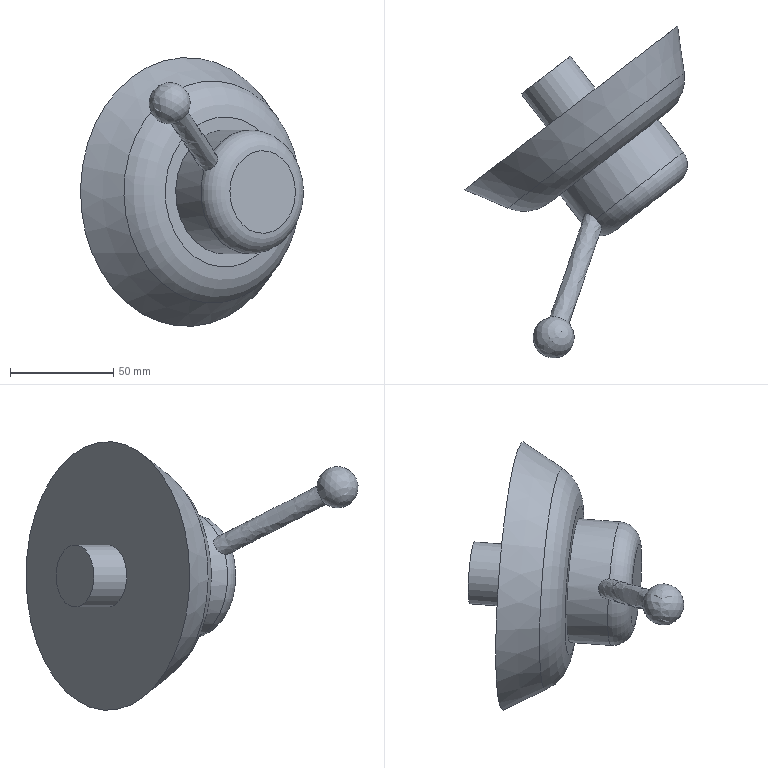Component | NX | BANSHOU2_2 | 1 solid | 11 faces | box 107.87 x 160.69 x 130 mm | volume 400459 mm3 | plane 4 | cylinder 2 | torus 2 | cone 1 | spline 1 | sphere 1 | commonest cylinder face diameters 30 x1 60 x1
STEP:
#1=CARTESIAN_POINT('',(0.,0.,0.));
#2=DIRECTION('',(0.,0.,1.));
#3=DIRECTION('',(1.,0.,0.));
#4=AXIS2_PLACEMENT_3D('',#1,#2,#3);
#5=CARTESIAN_POINT('',(170.195,-134.077,-526.));
#6=VERTEX_POINT('',#5);
#7=CARTESIAN_POINT('',(156.458,-144.627,-516.));
#8=DIRECTION('',(0.6091,-0.7931,0.));
#9=DIRECTION('',(0.6869,0.5275,-0.5));
#10=AXIS2_PLACEMENT_3D('',#7,#8,#9);
#11=CIRCLE('',#10,20.);
#12=CARTESIAN_POINT('',(170.195,-134.077,-526.));
#13=DIRECTION('',(-0.6091,0.7931,-0.));
#14=DIRECTION('',(-0.6869,-0.5275,0.5));
#15=AXIS2_PLACEMENT_3D('',#12,#13,#14);
#16=PLANE('',#15);
#17=CARTESIAN_POINT('',(-0.,-0.));
#18=CARTESIAN_POINT('',(-0.,34.641));
#19=CARTESIAN_POINT('',(30.,17.321));
#20=CARTESIAN_POINT('',(60.,0.));
#21=CARTESIAN_POINT('',(30.,-17.321));
#22=CARTESIAN_POINT('',(-0.,-34.641));
#23=CARTESIAN_POINT('',(-0.,-0.));
#24=(BOUNDED_CURVE()B_SPLINE_CURVE(2,(#17,#18,#19,#20,#21,#22,#23),.UNSPECIFIED.,.T.,.F.)B_SPLINE_CURVE_WITH_KNOTS((1,2,2,2,2,1),(-2.094,0.,2.094,4.189,6.283,8.378),.UNSPECIFIED.)CURVE()GEOMETRIC_REPRESENTATION_ITEM()RATIONAL_B_SPLINE_CURVE((1.,0.5,1.,0.5,1.,0.5,1.))REPRESENTATION_ITEM(''));
#25=(GEOMETRIC_REPRESENTATION_CONTEXT(2)PARAMETRIC_REPRESENTATION_CONTEXT()REPRESENTATION_CONTEXT('',''));
#26=DEFINITIONAL_REPRESENTATION('',(#24),#25);
#27=PCURVE('',#16,#26);
#28=CARTESIAN_POINT('',(150.367,-136.696,-516.));
#29=DIRECTION('',(0.6091,-0.7931,0.));
#30=DIRECTION('',(0.6869,0.5275,-0.5));
#31=AXIS2_PLACEMENT_3D('',#28,#29,#30);
#32=TOROIDAL_SURFACE('',#31,20.,10.);
#33=CARTESIAN_POINT('',(0.,7.854));
#34=DIRECTION('',(1.,0.));
#35=VECTOR('',#34,1.);
#36=LINE('',#33,#35);
#37=(GEOMETRIC_REPRESENTATION_CONTEXT(2)PARAMETRIC_REPRESENTATION_CONTEXT()REPRESENTATION_CONTEXT('',''));
#38=DEFINITIONAL_REPRESENTATION('',(#36),#37);
#39=PCURVE('',#32,#38);
#40=SURFACE_CURVE('',#11,(#27,#39),.PCURVE_S1.);
#41=EDGE_CURVE('',#6,#6,#40,.T.);
#42=ORIENTED_EDGE('',*,*,#41,.T.);
#43=EDGE_LOOP('',(#42));
#44=FACE_BOUND('',#43,.T.);
#45=ADVANCED_FACE('',(#44),#16,.F.);
#46=CARTESIAN_POINT('',(118.035,-73.266,-523.5));
#47=VERTEX_POINT('',#46);
#48=CARTESIAN_POINT('',(107.732,-81.178,-516.));
#49=DIRECTION('',(0.6091,-0.7931,0.));
#50=DIRECTION('',(0.6869,0.5275,-0.5));
#51=AXIS2_PLACEMENT_3D('',#48,#49,#50);
#52=CIRCLE('',#51,15.);
#53=CARTESIAN_POINT('',(107.732,-81.178,-516.));
#54=DIRECTION('',(0.6091,-0.7931,0.));
#55=DIRECTION('',(0.6869,0.5275,-0.5));
#56=AXIS2_PLACEMENT_3D('',#53,#54,#55);
#57=PLANE('',#56);
#58=CARTESIAN_POINT('',(0.,0.));
#59=DIRECTION('',(1.,-0.));
#60=AXIS2_PLACEMENT_2D('',#58,#59);
#61=CIRCLE('',#60,15.);
#62=(GEOMETRIC_REPRESENTATION_CONTEXT(2)PARAMETRIC_REPRESENTATION_CONTEXT()REPRESENTATION_CONTEXT('',''));
#63=DEFINITIONAL_REPRESENTATION('',(#61),#62);
#64=PCURVE('',#57,#63);
#65=CARTESIAN_POINT('',(119.913,-97.04,-516.));
#66=DIRECTION('',(0.6091,-0.7931,0.));
#67=DIRECTION('',(0.6869,0.5275,-0.5));
#68=AXIS2_PLACEMENT_3D('',#65,#66,#67);
#69=CYLINDRICAL_SURFACE('',#68,15.);
#70=CARTESIAN_POINT('',(0.,-20.));
#71=DIRECTION('',(1.,0.));
#72=VECTOR('',#71,1.);
#73=LINE('',#70,#72);
#74=(GEOMETRIC_REPRESENTATION_CONTEXT(2)PARAMETRIC_REPRESENTATION_CONTEXT()REPRESENTATION_CONTEXT('',''));
#75=DEFINITIONAL_REPRESENTATION('',(#73),#74);
#76=PCURVE('',#69,#75);
#77=SURFACE_CURVE('',#52,(#64,#76),.PCURVE_S1.);
#78=EDGE_CURVE('',#47,#47,#77,.T.);
#79=ORIENTED_EDGE('',*,*,#78,.F.);
#80=EDGE_LOOP('',(#79));
#81=FACE_BOUND('',#80,.T.);
#82=ADVANCED_FACE('',(#81),#57,.F.);
#83=CARTESIAN_POINT('',(130.216,-89.128,-523.5));
#84=VERTEX_POINT('',#83);
#85=CARTESIAN_POINT('',(119.913,-97.04,-516.));
#86=DIRECTION('',(0.6091,-0.7931,0.));
#87=DIRECTION('',(0.6869,0.5275,-0.5));
#88=AXIS2_PLACEMENT_3D('',#85,#86,#87);
#89=CIRCLE('',#88,15.);
#90=CARTESIAN_POINT('',(0.,0.));
#91=DIRECTION('',(1.,0.));
#92=VECTOR('',#91,1.);
#93=LINE('',#90,#92);
#94=(GEOMETRIC_REPRESENTATION_CONTEXT(2)PARAMETRIC_REPRESENTATION_CONTEXT()REPRESENTATION_CONTEXT('',''));
#95=DEFINITIONAL_REPRESENTATION('',(#93),#94);
#96=PCURVE('',#69,#95);
#97=CARTESIAN_POINT('',(130.216,-89.128,-523.5));
#98=DIRECTION('',(0.6091,-0.7931,0.));
#99=DIRECTION('',(0.6869,0.5275,-0.5));
#100=AXIS2_PLACEMENT_3D('',#97,#98,#99);
#101=PLANE('',#100);
#102=CARTESIAN_POINT('',(-15.,0.));
#103=DIRECTION('',(1.,-0.));
#104=AXIS2_PLACEMENT_2D('',#102,#103);
#105=CIRCLE('',#104,15.);
#106=(GEOMETRIC_REPRESENTATION_CONTEXT(2)PARAMETRIC_REPRESENTATION_CONTEXT()REPRESENTATION_CONTEXT('',''));
#107=DEFINITIONAL_REPRESENTATION('',(#105),#106);
#108=PCURVE('',#101,#107);
#109=SURFACE_CURVE('',#89,(#96,#108),.PCURVE_S1.);
#110=EDGE_CURVE('',#84,#84,#109,.T.);
#111=ORIENTED_EDGE('',*,*,#110,.F.);
#112=CARTESIAN_POINT('',(118.035,-73.266,-523.5));
#113=CARTESIAN_POINT('',(130.216,-89.128,-523.5));
#114=B_SPLINE_CURVE_WITH_KNOTS('',1,(#112,#113),.UNSPECIFIED.,.F.,.F.,(2,2),(-20.,0.),.PIECEWISE_BEZIER_KNOTS.);
#115=CARTESIAN_POINT('',(0.,0.));
#116=DIRECTION('',(0.,1.));
#117=VECTOR('',#116,1.);
#118=LINE('',#115,#117);
#119=(GEOMETRIC_REPRESENTATION_CONTEXT(2)PARAMETRIC_REPRESENTATION_CONTEXT()REPRESENTATION_CONTEXT('',''));
#120=DEFINITIONAL_REPRESENTATION('',(#118),#119);
#121=PCURVE('',#69,#120);
#122=CARTESIAN_POINT('',(6.283,0.));
#123=DIRECTION('',(0.,1.));
#124=VECTOR('',#123,1.);
#125=LINE('',#122,#124);
#126=(GEOMETRIC_REPRESENTATION_CONTEXT(2)PARAMETRIC_REPRESENTATION_CONTEXT()REPRESENTATION_CONTEXT('',''));
#127=DEFINITIONAL_REPRESENTATION('',(#125),#126);
#128=PCURVE('',#69,#127);
#129=SEAM_CURVE('',#114,(#121,#128),.PCURVE_S1.);
#130=EDGE_CURVE('',#47,#84,#129,.T.);
#131=ORIENTED_EDGE('',*,*,#130,.F.);
#132=ORIENTED_EDGE('',*,*,#78,.T.);
#133=ORIENTED_EDGE('',*,*,#130,.T.);
#134=EDGE_LOOP('',(#111,#131,#132,#133));
#135=FACE_BOUND('',#134,.T.);
#136=ADVANCED_FACE('',(#135),#69,.T.);
#137=CARTESIAN_POINT('',(164.559,-62.754,-548.5));
#138=VERTEX_POINT('',#137);
#139=CARTESIAN_POINT('',(119.913,-97.04,-516.));
#140=DIRECTION('',(0.6091,-0.7931,0.));
#141=DIRECTION('',(0.6869,0.5275,-0.5));
#142=AXIS2_PLACEMENT_3D('',#139,#140,#141);
#143=CIRCLE('',#142,65.);
#144=CARTESIAN_POINT('',(-15.,0.));
#145=DIRECTION('',(1.,0.));
#146=AXIS2_PLACEMENT_2D('',#144,#145);
#147=CIRCLE('',#146,65.);
#148=(GEOMETRIC_REPRESENTATION_CONTEXT(2)PARAMETRIC_REPRESENTATION_CONTEXT()REPRESENTATION_CONTEXT('',''));
#149=DEFINITIONAL_REPRESENTATION('',(#147),#148);
#150=PCURVE('',#101,#149);
#151=CARTESIAN_POINT('',(119.913,-97.04,-516.));
#152=DIRECTION('',(-0.6091,0.7931,-0.));
#153=DIRECTION('',(-0.6869,-0.5275,0.5));
#154=AXIS2_PLACEMENT_3D('',#151,#152,#153);
#155=CONICAL_SURFACE('',#154,65.,0.5155);
#156=CARTESIAN_POINT('',(9.425,0.));
#157=DIRECTION('',(-1.,0.));
#158=VECTOR('',#157,1.);
#159=LINE('',#156,#158);
#160=(GEOMETRIC_REPRESENTATION_CONTEXT(2)PARAMETRIC_REPRESENTATION_CONTEXT()REPRESENTATION_CONTEXT('',''));
#161=DEFINITIONAL_REPRESENTATION('',(#159),#160);
#162=PCURVE('',#155,#161);
#163=SURFACE_CURVE('',#143,(#150,#162),.PCURVE_S1.);
#164=EDGE_CURVE('',#138,#138,#163,.T.);
#165=ORIENTED_EDGE('',*,*,#164,.F.);
#166=EDGE_LOOP('',(#165));
#167=FACE_BOUND('',#166,.T.);
#168=ORIENTED_EDGE('',*,*,#110,.T.);
#169=EDGE_LOOP('',(#168));
#170=FACE_BOUND('',#169,.T.);
#171=ADVANCED_FACE('',(#167,#170),#101,.F.);
#172=CARTESIAN_POINT('',(168.925,-84.442,-542.873));
#173=VERTEX_POINT('',#172);
#174=CARTESIAN_POINT('',(132.01,-112.792,-516.));
#175=DIRECTION('',(0.6091,-0.7931,0.));
#176=DIRECTION('',(0.6869,0.5275,-0.5));
#177=AXIS2_PLACEMENT_3D('',#174,#175,#176);
#178=CIRCLE('',#177,53.746);
#179=CARTESIAN_POINT('',(9.425,-19.86));
#180=DIRECTION('',(-1.,0.));
#181=VECTOR('',#180,1.);
#182=LINE('',#179,#181);
#183=(GEOMETRIC_REPRESENTATION_CONTEXT(2)PARAMETRIC_REPRESENTATION_CONTEXT()REPRESENTATION_CONTEXT('',''));
#184=DEFINITIONAL_REPRESENTATION('',(#182),#183);
#185=PCURVE('',#155,#184);
#186=CARTESIAN_POINT('',(126.004,-104.971,-516.));
#187=DIRECTION('',(0.6091,-0.7931,0.));
#188=DIRECTION('',(0.6869,0.5275,-0.5));
#189=AXIS2_PLACEMENT_3D('',#186,#187,#188);
#190=TOROIDAL_SURFACE('',#189,36.345,20.);
#191=CARTESIAN_POINT('',(0.,6.799));
#192=DIRECTION('',(1.,0.));
#193=VECTOR('',#192,1.);
#194=LINE('',#191,#193);
#195=(GEOMETRIC_REPRESENTATION_CONTEXT(2)PARAMETRIC_REPRESENTATION_CONTEXT()REPRESENTATION_CONTEXT('',''));
#196=DEFINITIONAL_REPRESENTATION('',(#194),#195);
#197=PCURVE('',#190,#196);
#198=SURFACE_CURVE('',#178,(#185,#197),.PCURVE_S1.);
#199=EDGE_CURVE('',#173,#173,#198,.T.);
#200=ORIENTED_EDGE('',*,*,#199,.F.);
#201=CARTESIAN_POINT('',(168.925,-84.442,-542.873));
#202=CARTESIAN_POINT('',(164.559,-62.754,-548.5));
#203=B_SPLINE_CURVE_WITH_KNOTS('',1,(#201,#202),.UNSPECIFIED.,.F.,.F.,(2,2),(-22.827,0.),.PIECEWISE_BEZIER_KNOTS.);
#204=CARTESIAN_POINT('',(9.425,0.));
#205=DIRECTION('',(0.,1.));
#206=VECTOR('',#205,1.);
#207=LINE('',#204,#206);
#208=(GEOMETRIC_REPRESENTATION_CONTEXT(2)PARAMETRIC_REPRESENTATION_CONTEXT()REPRESENTATION_CONTEXT('',''));
#209=DEFINITIONAL_REPRESENTATION('',(#207),#208);
#210=PCURVE('',#155,#209);
#211=CARTESIAN_POINT('',(3.142,0.));
#212=DIRECTION('',(0.,1.));
#213=VECTOR('',#212,1.);
#214=LINE('',#211,#213);
#215=(GEOMETRIC_REPRESENTATION_CONTEXT(2)PARAMETRIC_REPRESENTATION_CONTEXT()REPRESENTATION_CONTEXT('',''));
#216=DEFINITIONAL_REPRESENTATION('',(#214),#215);
#217=PCURVE('',#155,#216);
#218=SEAM_CURVE('',#203,(#210,#217),.PCURVE_S1.);
#219=EDGE_CURVE('',#173,#138,#218,.T.);
#220=ORIENTED_EDGE('',*,*,#219,.T.);
#221=ORIENTED_EDGE('',*,*,#164,.T.);
#222=ORIENTED_EDGE('',*,*,#219,.F.);
#223=EDGE_LOOP('',(#200,#220,#221,#222));
#224=FACE_BOUND('',#223,.T.);
#225=ADVANCED_FACE('',(#224),#155,.T.);
#226=CARTESIAN_POINT('',(163.15,-101.662,-534.173));
#227=VERTEX_POINT('',#226);
#228=CARTESIAN_POINT('',(138.186,-120.834,-516.));
#229=DIRECTION('',(0.6091,-0.7931,0.));
#230=DIRECTION('',(0.6869,0.5275,-0.5));
#231=AXIS2_PLACEMENT_3D('',#228,#229,#230);
#232=CIRCLE('',#231,36.345);
#233=CARTESIAN_POINT('',(0.,7.854));
#234=DIRECTION('',(1.,0.));
#235=VECTOR('',#234,1.);
#236=LINE('',#233,#235);
#237=(GEOMETRIC_REPRESENTATION_CONTEXT(2)PARAMETRIC_REPRESENTATION_CONTEXT()REPRESENTATION_CONTEXT('',''));
#238=DEFINITIONAL_REPRESENTATION('',(#236),#237);
#239=PCURVE('',#190,#238);
#240=CARTESIAN_POINT('',(163.15,-101.662,-534.173));
#241=DIRECTION('',(-0.6091,0.7931,-0.));
#242=DIRECTION('',(-0.6869,-0.5275,0.5));
#243=AXIS2_PLACEMENT_3D('',#240,#241,#242);
#244=PLANE('',#243);
#245=CARTESIAN_POINT('',(-0.,0.));
#246=CARTESIAN_POINT('',(-0.,62.952));
#247=CARTESIAN_POINT('',(54.518,31.476));
#248=CARTESIAN_POINT('',(109.036,0.));
#249=CARTESIAN_POINT('',(54.518,-31.476));
#250=CARTESIAN_POINT('',(-0.,-62.952));
#251=CARTESIAN_POINT('',(-0.,0.));
#252=(BOUNDED_CURVE()B_SPLINE_CURVE(2,(#245,#246,#247,#248,#249,#250,#251),.UNSPECIFIED.,.T.,.F.)B_SPLINE_CURVE_WITH_KNOTS((1,2,2,2,2,1),(-2.094,0.,2.094,4.189,6.283,8.378),.UNSPECIFIED.)CURVE()GEOMETRIC_REPRESENTATION_ITEM()RATIONAL_B_SPLINE_CURVE((1.,0.5,1.,0.5,1.,0.5,1.))REPRESENTATION_ITEM(''));
#253=(GEOMETRIC_REPRESENTATION_CONTEXT(2)PARAMETRIC_REPRESENTATION_CONTEXT()REPRESENTATION_CONTEXT('',''));
#254=DEFINITIONAL_REPRESENTATION('',(#252),#253);
#255=PCURVE('',#244,#254);
#256=SURFACE_CURVE('',#232,(#239,#255),.PCURVE_S1.);
#257=EDGE_CURVE('',#227,#227,#256,.T.);
#258=ORIENTED_EDGE('',*,*,#257,.F.);
#259=CARTESIAN_POINT('',(168.925,-84.442,-542.873));
#260=CARTESIAN_POINT('',(169.605,-87.815,-541.998));
#261=CARTESIAN_POINT('',(169.599,-91.201,-540.805));
#262=CARTESIAN_POINT('',(168.901,-94.43,-539.349));
#263=CARTESIAN_POINT('',(167.54,-97.34,-537.703));
#264=CARTESIAN_POINT('',(165.588,-99.789,-535.948));
#265=CARTESIAN_POINT('',(163.15,-101.662,-534.173));
#266=(BOUNDED_CURVE()B_SPLINE_CURVE(6,(#259,#260,#261,#262,#263,#264,#265),.UNSPECIFIED.,.F.,.F.)B_SPLINE_CURVE_WITH_KNOTS((7,7),(0.5155,1.571),.PIECEWISE_BEZIER_KNOTS.)CURVE()GEOMETRIC_REPRESENTATION_ITEM()RATIONAL_B_SPLINE_CURVE((1.014,1.005,0.9991,0.9972,0.9991,1.005,1.014))REPRESENTATION_ITEM(''));
#267=CARTESIAN_POINT('',(0.,6.283));
#268=DIRECTION('',(0.,1.));
#269=VECTOR('',#268,1.);
#270=LINE('',#267,#269);
#271=(GEOMETRIC_REPRESENTATION_CONTEXT(2)PARAMETRIC_REPRESENTATION_CONTEXT()REPRESENTATION_CONTEXT('',''));
#272=DEFINITIONAL_REPRESENTATION('',(#270),#271);
#273=PCURVE('',#190,#272);
#274=CARTESIAN_POINT('',(6.283,6.283));
#275=DIRECTION('',(0.,1.));
#276=VECTOR('',#275,1.);
#277=LINE('',#274,#276);
#278=(GEOMETRIC_REPRESENTATION_CONTEXT(2)PARAMETRIC_REPRESENTATION_CONTEXT()REPRESENTATION_CONTEXT('',''));
#279=DEFINITIONAL_REPRESENTATION('',(#277),#278);
#280=PCURVE('',#190,#279);
#281=SEAM_CURVE('',#266,(#273,#280),.PCURVE_S1.);
#282=EDGE_CURVE('',#173,#227,#281,.T.);
#283=ORIENTED_EDGE('',*,*,#282,.F.);
#284=ORIENTED_EDGE('',*,*,#199,.T.);
#285=ORIENTED_EDGE('',*,*,#282,.T.);
#286=EDGE_LOOP('',(#258,#283,#284,#285));
#287=FACE_BOUND('',#286,.T.);
#288=ADVANCED_FACE('',(#287),#190,.T.);
#289=CARTESIAN_POINT('',(158.791,-105.009,-531.));
#290=VERTEX_POINT('',#289);
#291=CARTESIAN_POINT('',(138.186,-120.834,-516.));
#292=DIRECTION('',(0.6091,-0.7931,0.));
#293=DIRECTION('',(0.6869,0.5275,-0.5));
#294=AXIS2_PLACEMENT_3D('',#291,#292,#293);
#295=CIRCLE('',#294,30.);
#296=CARTESIAN_POINT('',(6.345,0.));
#297=CARTESIAN_POINT('',(6.345,51.962));
#298=CARTESIAN_POINT('',(51.345,25.981));
#299=CARTESIAN_POINT('',(96.345,0.));
#300=CARTESIAN_POINT('',(51.345,-25.981));
#301=CARTESIAN_POINT('',(6.345,-51.962));
#302=CARTESIAN_POINT('',(6.345,0.));
#303=(BOUNDED_CURVE()B_SPLINE_CURVE(2,(#296,#297,#298,#299,#300,#301,#302),.UNSPECIFIED.,.T.,.F.)B_SPLINE_CURVE_WITH_KNOTS((1,2,2,2,2,1),(-2.094,0.,2.094,4.189,6.283,8.378),.UNSPECIFIED.)CURVE()GEOMETRIC_REPRESENTATION_ITEM()RATIONAL_B_SPLINE_CURVE((1.,0.5,1.,0.5,1.,0.5,1.))REPRESENTATION_ITEM(''));
#304=(GEOMETRIC_REPRESENTATION_CONTEXT(2)PARAMETRIC_REPRESENTATION_CONTEXT()REPRESENTATION_CONTEXT('',''));
#305=DEFINITIONAL_REPRESENTATION('',(#303),#304);
#306=PCURVE('',#244,#305);
#307=CARTESIAN_POINT('',(119.913,-97.04,-516.));
#308=DIRECTION('',(0.6091,-0.7931,0.));
#309=DIRECTION('',(0.6869,0.5275,-0.5));
#310=AXIS2_PLACEMENT_3D('',#307,#308,#309);
#311=CYLINDRICAL_SURFACE('',#310,30.);
#312=CARTESIAN_POINT('',(0.,30.));
#313=DIRECTION('',(1.,0.));
#314=VECTOR('',#313,1.);
#315=LINE('',#312,#314);
#316=(GEOMETRIC_REPRESENTATION_CONTEXT(2)PARAMETRIC_REPRESENTATION_CONTEXT()REPRESENTATION_CONTEXT('',''));
#317=DEFINITIONAL_REPRESENTATION('',(#315),#316);
#318=PCURVE('',#311,#317);
#319=SURFACE_CURVE('',#295,(#306,#318),.PCURVE_S1.);
#320=EDGE_CURVE('',#290,#290,#319,.T.);
#321=ORIENTED_EDGE('',*,*,#320,.F.);
#322=EDGE_LOOP('',(#321));
#323=FACE_BOUND('',#322,.T.);
#324=ORIENTED_EDGE('',*,*,#257,.T.);
#325=EDGE_LOOP('',(#324));
#326=FACE_BOUND('',#325,.T.);
#327=ADVANCED_FACE('',(#323,#326),#244,.F.);
#328=CARTESIAN_POINT('',(170.973,-120.872,-531.));
#329=VERTEX_POINT('',#328);
#330=CARTESIAN_POINT('',(132.021,-150.784,-496.896));
#331=VERTEX_POINT('',#330);
#332=CARTESIAN_POINT('',(150.367,-136.696,-516.));
#333=DIRECTION('',(0.6091,-0.7931,0.));
#334=DIRECTION('',(0.6869,0.5275,-0.5));
#335=AXIS2_PLACEMENT_3D('',#332,#333,#334);
#336=CIRCLE('',#335,30.);
#337=CARTESIAN_POINT('',(-6.283,50.));
#338=DIRECTION('',(1.,0.));
#339=VECTOR('',#338,1.);
#340=LINE('',#337,#339);
#341=(GEOMETRIC_REPRESENTATION_CONTEXT(2)PARAMETRIC_REPRESENTATION_CONTEXT()REPRESENTATION_CONTEXT('',''));
#342=DEFINITIONAL_REPRESENTATION('',(#340),#341);
#343=PCURVE('',#311,#342);
#344=CARTESIAN_POINT('',(-6.283,6.283));
#345=DIRECTION('',(1.,0.));
#346=VECTOR('',#345,1.);
#347=LINE('',#344,#346);
#348=(GEOMETRIC_REPRESENTATION_CONTEXT(2)PARAMETRIC_REPRESENTATION_CONTEXT()REPRESENTATION_CONTEXT('',''));
#349=DEFINITIONAL_REPRESENTATION('',(#347),#348);
#350=PCURVE('',#32,#349);
#351=SURFACE_CURVE('',#336,(#343,#350),.PCURVE_S1.);
#352=EDGE_CURVE('',#329,#331,#351,.T.);
#353=ORIENTED_EDGE('',*,*,#352,.F.);
#354=CARTESIAN_POINT('',(158.791,-105.009,-531.));
#355=CARTESIAN_POINT('',(170.973,-120.872,-531.));
#356=B_SPLINE_CURVE_WITH_KNOTS('',1,(#354,#355),.UNSPECIFIED.,.F.,.F.,(2,2),(30.,50.),.PIECEWISE_BEZIER_KNOTS.);
#357=CARTESIAN_POINT('',(0.,0.));
#358=DIRECTION('',(0.,1.));
#359=VECTOR('',#358,1.);
#360=LINE('',#357,#359);
#361=(GEOMETRIC_REPRESENTATION_CONTEXT(2)PARAMETRIC_REPRESENTATION_CONTEXT()REPRESENTATION_CONTEXT('',''));
#362=DEFINITIONAL_REPRESENTATION('',(#360),#361);
#363=PCURVE('',#311,#362);
#364=CARTESIAN_POINT('',(6.283,0.));
#365=DIRECTION('',(0.,1.));
#366=VECTOR('',#365,1.);
#367=LINE('',#364,#366);
#368=(GEOMETRIC_REPRESENTATION_CONTEXT(2)PARAMETRIC_REPRESENTATION_CONTEXT()REPRESENTATION_CONTEXT('',''));
#369=DEFINITIONAL_REPRESENTATION('',(#367),#368);
#370=PCURVE('',#311,#369);
#371=SEAM_CURVE('',#356,(#363,#370),.PCURVE_S1.);
#372=EDGE_CURVE('',#290,#329,#371,.T.);
#373=ORIENTED_EDGE('',*,*,#372,.F.);
#374=ORIENTED_EDGE('',*,*,#320,.T.);
#375=ORIENTED_EDGE('',*,*,#372,.T.);
#376=CARTESIAN_POINT('',(128.073,-153.817,-505.52));
#377=VERTEX_POINT('',#376);
#378=CARTESIAN_POINT('',(150.367,-136.696,-516.));
#379=DIRECTION('',(0.6091,-0.7931,0.));
#380=DIRECTION('',(0.6869,0.5275,-0.5));
#381=AXIS2_PLACEMENT_3D('',#378,#379,#380);
#382=CIRCLE('',#381,30.);
#383=CARTESIAN_POINT('',(0.,50.));
#384=DIRECTION('',(1.,0.));
#385=VECTOR('',#384,1.);
#386=LINE('',#383,#385);
#387=(GEOMETRIC_REPRESENTATION_CONTEXT(2)PARAMETRIC_REPRESENTATION_CONTEXT()REPRESENTATION_CONTEXT('',''));
#388=DEFINITIONAL_REPRESENTATION('',(#386),#387);
#389=PCURVE('',#311,#388);
#390=CARTESIAN_POINT('',(-0.,6.283));
#391=DIRECTION('',(1.,0.));
#392=VECTOR('',#391,1.);
#393=LINE('',#390,#392);
#394=(GEOMETRIC_REPRESENTATION_CONTEXT(2)PARAMETRIC_REPRESENTATION_CONTEXT()REPRESENTATION_CONTEXT('',''));
#395=DEFINITIONAL_REPRESENTATION('',(#393),#394);
#396=PCURVE('',#32,#395);
#397=SURFACE_CURVE('',#382,(#389,#396),.PCURVE_S1.);
#398=EDGE_CURVE('',#377,#329,#397,.T.);
#399=ORIENTED_EDGE('',*,*,#398,.F.);
#400=CARTESIAN_POINT('',(128.073,-153.817,-505.52));
#401=CARTESIAN_POINT('',(127.309,-152.761,-505.419));
#402=CARTESIAN_POINT('',(126.684,-151.667,-504.941));
#403=CARTESIAN_POINT('',(126.105,-149.738,-503.283));
#404=CARTESIAN_POINT('',(126.199,-148.955,-502.134));
#405=CARTESIAN_POINT('',(127.226,-148.16,-499.883));
#406=CARTESIAN_POINT('',(128.145,-148.167,-498.822));
#407=CARTESIAN_POINT('',(130.132,-148.991,-497.378));
#408=CARTESIAN_POINT('',(131.173,-149.792,-496.979));
#409=CARTESIAN_POINT('',(132.021,-150.784,-496.896));
#410=B_SPLINE_CURVE_WITH_KNOTS('',3,(#400,#401,#402,#403,#404,#405,#406,#407,#408,#409),.UNSPECIFIED.,.F.,.F.,(4,2,2,2,4),(0.,0.25,0.5,0.75,1.),.UNSPECIFIED.);
#411=CARTESIAN_POINT('',(3.308,50.));
#412=CARTESIAN_POINT('',(3.308,49.763));
#413=CARTESIAN_POINT('',(3.305,49.293));
#414=CARTESIAN_POINT('',(3.3,48.608));
#415=CARTESIAN_POINT('',(3.291,47.952));
#416=CARTESIAN_POINT('',(3.28,47.333));
#417=CARTESIAN_POINT('',(3.266,46.763));
#418=CARTESIAN_POINT('',(3.25,46.247));
#419=CARTESIAN_POINT('',(3.231,45.811));
#420=CARTESIAN_POINT('',(3.21,45.46));
#421=CARTESIAN_POINT('',(3.188,45.2));
#422=CARTESIAN_POINT('',(3.165,45.039));
#423=CARTESIAN_POINT('',(3.142,44.981));
#424=CARTESIAN_POINT('',(3.118,45.036));
#425=CARTESIAN_POINT('',(3.095,45.197));
#426=CARTESIAN_POINT('',(3.073,45.455));
#427=CARTESIAN_POINT('',(3.053,45.805));
#428=CARTESIAN_POINT('',(3.034,46.237));
#429=CARTESIAN_POINT('',(3.018,46.747));
#430=CARTESIAN_POINT('',(3.004,47.318));
#431=CARTESIAN_POINT('',(2.992,47.94));
#432=CARTESIAN_POINT('',(2.984,48.601));
#433=CARTESIAN_POINT('',(2.978,49.291));
#434=CARTESIAN_POINT('',(2.976,49.763));
#435=CARTESIAN_POINT('',(2.975,50.));
#436=B_SPLINE_CURVE_WITH_KNOTS('',3,(#411,#412,#413,#414,#415,#416,#417,#418,#419,#420,#421,#422,#423,#424,#425,#426,#427,#428,#429,#430,#431,#432,#433,#434,#435),.UNSPECIFIED.,.F.,.F.,(4,1,1,1,1,1,1,1,1,1,1,1,1,1,1,1,1,1,1,1,1,1,4),(0.,0.04545,0.09091,0.1364,0.1818,0.2273,0.2727,0.3182,0.3636,0.4091,0.4545,0.5,0.5455,0.5909,0.6364,0.6818,0.7273,0.7727,0.8182,0.8636,0.9091,0.9545,1.),.QUASI_UNIFORM_KNOTS.);
#437=(GEOMETRIC_REPRESENTATION_CONTEXT(2)PARAMETRIC_REPRESENTATION_CONTEXT()REPRESENTATION_CONTEXT('',''));
#438=DEFINITIONAL_REPRESENTATION('',(#436),#437);
#439=PCURVE('',#311,#438);
#440=CARTESIAN_POINT('',(134.905,-152.793,-505.3));
#441=CARTESIAN_POINT('',(125.04,-181.791,-490.586));
#442=CARTESIAN_POINT('',(115.176,-210.789,-475.872));
#443=CARTESIAN_POINT('',(136.307,-151.717,-502.238));
#444=CARTESIAN_POINT('',(126.442,-180.715,-487.524));
#445=CARTESIAN_POINT('',(116.578,-209.712,-472.81));
#446=CARTESIAN_POINT('',(136.468,-150.628,-499.984));
#447=CARTESIAN_POINT('',(126.604,-179.625,-485.27));
#448=CARTESIAN_POINT('',(116.739,-208.623,-470.555));
#449=CARTESIAN_POINT('',(134.773,-149.365,-498.631));
#450=CARTESIAN_POINT('',(124.909,-178.363,-483.917));
#451=CARTESIAN_POINT('',(115.044,-207.361,-469.203));
#452=CARTESIAN_POINT('',(131.694,-147.869,-497.747));
#453=CARTESIAN_POINT('',(121.83,-176.867,-483.033));
#454=CARTESIAN_POINT('',(111.965,-205.865,-468.319));
#455=CARTESIAN_POINT('',(129.299,-147.144,-497.926));
#456=CARTESIAN_POINT('',(119.434,-176.142,-483.211));
#457=CARTESIAN_POINT('',(109.57,-205.14,-468.497));
#458=CARTESIAN_POINT('',(127.598,-147.485,-499.738));
#459=CARTESIAN_POINT('',(117.733,-176.483,-485.024));
#460=CARTESIAN_POINT('',(107.869,-205.481,-470.31));
#461=CARTESIAN_POINT('',(126.196,-148.562,-502.8));
#462=CARTESIAN_POINT('',(116.331,-177.56,-488.086));
#463=CARTESIAN_POINT('',(106.467,-206.558,-473.372));
#464=CARTESIAN_POINT('',(126.034,-149.651,-505.055));
#465=CARTESIAN_POINT('',(116.17,-178.649,-490.341));
#466=CARTESIAN_POINT('',(106.305,-207.647,-475.627));
#467=CARTESIAN_POINT('',(127.729,-150.914,-506.407));
#468=CARTESIAN_POINT('',(117.864,-179.912,-491.693));
#469=CARTESIAN_POINT('',(108.,-208.91,-476.979));
#470=CARTESIAN_POINT('',(130.808,-152.41,-507.291));
#471=CARTESIAN_POINT('',(120.943,-181.408,-492.577));
#472=CARTESIAN_POINT('',(111.079,-210.406,-477.863));
#473=CARTESIAN_POINT('',(133.204,-153.135,-507.113));
#474=CARTESIAN_POINT('',(123.339,-182.132,-492.399));
#475=CARTESIAN_POINT('',(113.475,-211.13,-477.685));
#476=CARTESIAN_POINT('',(134.905,-152.793,-505.3));
#477=CARTESIAN_POINT('',(125.04,-181.791,-490.586));
#478=CARTESIAN_POINT('',(115.176,-210.789,-475.872));
#479=CARTESIAN_POINT('',(136.307,-151.717,-502.238));
#480=CARTESIAN_POINT('',(126.442,-180.715,-487.524));
#481=CARTESIAN_POINT('',(116.578,-209.712,-472.81));
#482=(BOUNDED_SURFACE()B_SPLINE_SURFACE(4,2,((#440,#441,#442),(#443,#444,#445),(#446,#447,#448),(#449,#450,#451),(#452,#453,#454),(#455,#456,#457),(#458,#459,#460),(#461,#462,#463),(#464,#465,#466),(#467,#468,#469),(#470,#471,#472),(#473,#474,#475),(#476,#477,#478),(#479,#480,#481)),.UNSPECIFIED.,.T.,.F.,.F.)B_SPLINE_SURFACE_WITH_KNOTS((2,3,3,3,3,3,2),(3,3),(-0.25,0.,0.25,0.5,0.75,1.,1.25),(0.,1.),.UNSPECIFIED.)GEOMETRIC_REPRESENTATION_ITEM()RATIONAL_B_SPLINE_SURFACE(((0.5858,0.5858,0.5858),(0.5858,0.5858,0.5858),(0.5523,0.5523,0.5523),(0.5858,0.5858,0.5858),(0.5858,0.5858,0.5858),(0.5523,0.5523,0.5523),(0.5858,0.5858,0.5858),(0.5858,0.5858,0.5858),(0.5523,0.5523,0.5523),(0.5858,0.5858,0.5858),(0.5858,0.5858,0.5858),(0.5523,0.5523,0.5523),(0.5858,0.5858,0.5858),(0.5858,0.5858,0.5858)))REPRESENTATION_ITEM('')SURFACE());
#483=CARTESIAN_POINT('',(0.7339,0.04063));
#484=CARTESIAN_POINT('',(0.7269,0.03893));
#485=CARTESIAN_POINT('',(0.713,0.03562));
#486=CARTESIAN_POINT('',(0.6927,0.03095));
#487=CARTESIAN_POINT('',(0.6727,0.02663));
#488=CARTESIAN_POINT('',(0.6528,0.02269));
#489=CARTESIAN_POINT('',(0.6328,0.01917));
#490=CARTESIAN_POINT('',(0.6123,0.01612));
#491=CARTESIAN_POINT('',(0.5914,0.0136));
#492=CARTESIAN_POINT('',(0.57,0.01163));
#493=CARTESIAN_POINT('',(0.5478,0.01021));
#494=CARTESIAN_POINT('',(0.5249,0.009348));
#495=CARTESIAN_POINT('',(0.5004,0.009053));
#496=CARTESIAN_POINT('',(0.4757,0.009335));
#497=CARTESIAN_POINT('',(0.4527,0.01019));
#498=CARTESIAN_POINT('',(0.4305,0.0116));
#499=CARTESIAN_POINT('',(0.409,0.01356));
#500=CARTESIAN_POINT('',(0.3882,0.01606));
#501=CARTESIAN_POINT('',(0.3678,0.01908));
#502=CARTESIAN_POINT('',(0.3477,0.0226));
#503=CARTESIAN_POINT('',(0.3277,0.02656));
#504=CARTESIAN_POINT('',(0.3076,0.03091));
#505=CARTESIAN_POINT('',(0.2871,0.03561));
#506=CARTESIAN_POINT('',(0.2731,0.03893));
#507=CARTESIAN_POINT('',(0.2661,0.04063));
#508=B_SPLINE_CURVE_WITH_KNOTS('',3,(#483,#484,#485,#486,#487,#488,#489,#490,#491,#492,#493,#494,#495,#496,#497,#498,#499,#500,#501,#502,#503,#504,#505,#506,#507),.UNSPECIFIED.,.F.,.F.,(4,1,1,1,1,1,1,1,1,1,1,1,1,1,1,1,1,1,1,1,1,1,4),(0.,0.04545,0.09091,0.1364,0.1818,0.2273,0.2727,0.3182,0.3636,0.4091,0.4545,0.5,0.5455,0.5909,0.6364,0.6818,0.7273,0.7727,0.8182,0.8636,0.9091,0.9545,1.),.QUASI_UNIFORM_KNOTS.);
#509=(GEOMETRIC_REPRESENTATION_CONTEXT(2)PARAMETRIC_REPRESENTATION_CONTEXT()REPRESENTATION_CONTEXT('',''));
#510=DEFINITIONAL_REPRESENTATION('',(#508),#509);
#511=PCURVE('',#482,#510);
#512=SURFACE_CURVE('',#410,(#439,#511),.PCURVE_S1.);
#513=EDGE_CURVE('',#377,#331,#512,.T.);
#514=ORIENTED_EDGE('',*,*,#513,.T.);
#515=EDGE_LOOP('',(#353,#373,#374,#375,#399,#514));
#516=FACE_BOUND('',#515,.T.);
#517=ADVANCED_FACE('',(#516),#311,.T.);
#518=ORIENTED_EDGE('',*,*,#41,.F.);
#519=CARTESIAN_POINT('',(170.973,-120.872,-531.));
#520=CARTESIAN_POINT('',(172.601,-122.992,-531.));
#521=CARTESIAN_POINT('',(173.603,-125.505,-530.575));
#522=CARTESIAN_POINT('',(173.849,-128.144,-529.76));
#523=CARTESIAN_POINT('',(173.302,-130.62,-528.639));
#524=CARTESIAN_POINT('',(172.031,-132.667,-527.337));
#525=CARTESIAN_POINT('',(170.195,-134.077,-526.));
#526=(BOUNDED_CURVE()B_SPLINE_CURVE(6,(#519,#520,#521,#522,#523,#524,#525),.UNSPECIFIED.,.F.,.F.)B_SPLINE_CURVE_WITH_KNOTS((7,7),(0.,1.571),.PIECEWISE_BEZIER_KNOTS.)CURVE()GEOMETRIC_REPRESENTATION_ITEM()RATIONAL_B_SPLINE_CURVE((1.031,1.01,0.9979,0.994,0.9979,1.01,1.031))REPRESENTATION_ITEM(''));
#527=CARTESIAN_POINT('',(0.,6.283));
#528=DIRECTION('',(0.,1.));
#529=VECTOR('',#528,1.);
#530=LINE('',#527,#529);
#531=(GEOMETRIC_REPRESENTATION_CONTEXT(2)PARAMETRIC_REPRESENTATION_CONTEXT()REPRESENTATION_CONTEXT('',''));
#532=DEFINITIONAL_REPRESENTATION('',(#530),#531);
#533=PCURVE('',#32,#532);
#534=CARTESIAN_POINT('',(6.283,6.283));
#535=DIRECTION('',(0.,1.));
#536=VECTOR('',#535,1.);
#537=LINE('',#534,#536);
#538=(GEOMETRIC_REPRESENTATION_CONTEXT(2)PARAMETRIC_REPRESENTATION_CONTEXT()REPRESENTATION_CONTEXT('',''));
#539=DEFINITIONAL_REPRESENTATION('',(#537),#538);
#540=PCURVE('',#32,#539);
#541=SEAM_CURVE('',#526,(#533,#540),.PCURVE_S1.);
#542=EDGE_CURVE('',#329,#6,#541,.T.);
#543=ORIENTED_EDGE('',*,*,#542,.F.);
#544=ORIENTED_EDGE('',*,*,#352,.T.);
#545=CARTESIAN_POINT('',(134.317,-156.043,-501.847));
#546=VERTEX_POINT('',#545);
#547=CARTESIAN_POINT('',(132.021,-150.784,-496.896));
#548=CARTESIAN_POINT('',(132.957,-151.879,-496.805));
#549=CARTESIAN_POINT('',(133.893,-153.008,-497.292));
#550=CARTESIAN_POINT('',(134.88,-154.868,-499.214));
#551=CARTESIAN_POINT('',(134.891,-155.601,-500.592));
#552=CARTESIAN_POINT('',(133.747,-156.483,-503.095));
#553=CARTESIAN_POINT('',(132.618,-156.611,-504.165));
#554=CARTESIAN_POINT('',(130.173,-155.875,-505.432));
#555=CARTESIAN_POINT('',(128.917,-154.983,-505.63));
#556=CARTESIAN_POINT('',(128.073,-153.817,-505.52));
#557=B_SPLINE_CURVE_WITH_KNOTS('',3,(#547,#548,#549,#550,#551,#552,#553,#554,#555,#556),.UNSPECIFIED.,.F.,.F.,(4,2,2,2,4),(0.,0.25,0.5,0.75,1.),.UNSPECIFIED.);
#558=CARTESIAN_POINT('',(2.975,6.283));
#559=CARTESIAN_POINT('',(2.974,6.309));
#560=CARTESIAN_POINT('',(2.974,6.362));
#561=CARTESIAN_POINT('',(2.976,6.44));
#562=CARTESIAN_POINT('',(2.982,6.516));
#563=CARTESIAN_POINT('',(2.991,6.589));
#564=CARTESIAN_POINT('',(3.003,6.658));
#565=CARTESIAN_POINT('',(3.02,6.72));
#566=CARTESIAN_POINT('',(3.039,6.773));
#567=CARTESIAN_POINT('',(3.062,6.816));
#568=CARTESIAN_POINT('',(3.087,6.849));
#569=CARTESIAN_POINT('',(3.114,6.869));
#570=CARTESIAN_POINT('',(3.141,6.876));
#571=CARTESIAN_POINT('',(3.169,6.869));
#572=CARTESIAN_POINT('',(3.196,6.849));
#573=CARTESIAN_POINT('',(3.221,6.816));
#574=CARTESIAN_POINT('',(3.244,6.773));
#575=CARTESIAN_POINT('',(3.263,6.72));
#576=CARTESIAN_POINT('',(3.28,6.658));
#577=CARTESIAN_POINT('',(3.292,6.59));
#578=CARTESIAN_POINT('',(3.301,6.517));
#579=CARTESIAN_POINT('',(3.307,6.44));
#580=CARTESIAN_POINT('',(3.309,6.362));
#581=CARTESIAN_POINT('',(3.309,6.309));
#582=CARTESIAN_POINT('',(3.308,6.283));
#583=B_SPLINE_CURVE_WITH_KNOTS('',3,(#558,#559,#560,#561,#562,#563,#564,#565,#566,#567,#568,#569,#570,#571,#572,#573,#574,#575,#576,#577,#578,#579,#580,#581,#582),.UNSPECIFIED.,.F.,.F.,(4,1,1,1,1,1,1,1,1,1,1,1,1,1,1,1,1,1,1,1,1,1,4),(0.,0.04545,0.09091,0.1364,0.1818,0.2273,0.2727,0.3182,0.3636,0.4091,0.4545,0.5,0.5455,0.5909,0.6364,0.6818,0.7273,0.7727,0.8182,0.8636,0.9091,0.9545,1.),.QUASI_UNIFORM_KNOTS.);
#584=(GEOMETRIC_REPRESENTATION_CONTEXT(2)PARAMETRIC_REPRESENTATION_CONTEXT()REPRESENTATION_CONTEXT('',''));
#585=DEFINITIONAL_REPRESENTATION('',(#583),#584);
#586=PCURVE('',#32,#585);
#587=CARTESIAN_POINT('',(0.2661,0.04063));
#588=CARTESIAN_POINT('',(0.258,0.04251));
#589=CARTESIAN_POINT('',(0.2417,0.04605));
#590=CARTESIAN_POINT('',(0.2174,0.05071));
#591=CARTESIAN_POINT('',(0.1937,0.05469));
#592=CARTESIAN_POINT('',(0.1705,0.05798));
#593=CARTESIAN_POINT('',(0.1475,0.06057));
#594=CARTESIAN_POINT('',(0.1243,0.06244));
#595=CARTESIAN_POINT('',(0.101,0.06375));
#596=CARTESIAN_POINT('',(0.07727,0.0646));
#597=CARTESIAN_POINT('',(0.05277,0.06508));
#598=CARTESIAN_POINT('',(0.02742,0.06529));
#599=CARTESIAN_POINT('',(0.0001557,0.06533));
#600=CARTESIAN_POINT('',(-0.02714,0.06529));
#601=CARTESIAN_POINT('',(-0.0525,0.06508));
#602=CARTESIAN_POINT('',(-0.077,0.06461));
#603=CARTESIAN_POINT('',(-0.1008,0.06376));
#604=CARTESIAN_POINT('',(-0.1241,0.06246));
#605=CARTESIAN_POINT('',(-0.1472,0.0606));
#606=CARTESIAN_POINT('',(-0.1702,0.058));
#607=CARTESIAN_POINT('',(-0.1936,0.05471));
#608=CARTESIAN_POINT('',(-0.2173,0.05072));
#609=CARTESIAN_POINT('',(-0.2417,0.04606));
#610=CARTESIAN_POINT('',(-0.258,0.04251));
#611=CARTESIAN_POINT('',(-0.2661,0.04063));
#612=B_SPLINE_CURVE_WITH_KNOTS('',3,(#587,#588,#589,#590,#591,#592,#593,#594,#595,#596,#597,#598,#599,#600,#601,#602,#603,#604,#605,#606,#607,#608,#609,#610,#611),.UNSPECIFIED.,.F.,.F.,(4,1,1,1,1,1,1,1,1,1,1,1,1,1,1,1,1,1,1,1,1,1,4),(0.,0.04545,0.09091,0.1364,0.1818,0.2273,0.2727,0.3182,0.3636,0.4091,0.4545,0.5,0.5455,0.5909,0.6364,0.6818,0.7273,0.7727,0.8182,0.8636,0.9091,0.9545,1.),.QUASI_UNIFORM_KNOTS.);
#613=(GEOMETRIC_REPRESENTATION_CONTEXT(2)PARAMETRIC_REPRESENTATION_CONTEXT()REPRESENTATION_CONTEXT('',''));
#614=DEFINITIONAL_REPRESENTATION('',(#612),#613);
#615=PCURVE('',#482,#614);
#616=SURFACE_CURVE('',#557,(#586,#615),.PCURVE_S1.);
#617=EDGE_CURVE('',#331,#546,#616,.T.);
#618=ORIENTED_EDGE('',*,*,#617,.T.);
#619=CARTESIAN_POINT('',(132.021,-150.784,-496.896));
#620=CARTESIAN_POINT('',(132.957,-151.879,-496.805));
#621=CARTESIAN_POINT('',(133.893,-153.008,-497.292));
#622=CARTESIAN_POINT('',(134.88,-154.868,-499.214));
#623=CARTESIAN_POINT('',(134.891,-155.601,-500.592));
#624=CARTESIAN_POINT('',(133.747,-156.483,-503.095));
#625=CARTESIAN_POINT('',(132.618,-156.611,-504.165));
#626=CARTESIAN_POINT('',(130.173,-155.875,-505.432));
#627=CARTESIAN_POINT('',(128.917,-154.983,-505.63));
#628=CARTESIAN_POINT('',(128.073,-153.817,-505.52));
#629=B_SPLINE_CURVE_WITH_KNOTS('',3,(#619,#620,#621,#622,#623,#624,#625,#626,#627,#628),.UNSPECIFIED.,.F.,.F.,(4,2,2,2,4),(0.,0.25,0.5,0.75,1.),.UNSPECIFIED.);
#630=CARTESIAN_POINT('',(2.975,6.283));
#631=CARTESIAN_POINT('',(2.974,6.309));
#632=CARTESIAN_POINT('',(2.974,6.362));
#633=CARTESIAN_POINT('',(2.976,6.44));
#634=CARTESIAN_POINT('',(2.982,6.516));
#635=CARTESIAN_POINT('',(2.991,6.589));
#636=CARTESIAN_POINT('',(3.003,6.658));
#637=CARTESIAN_POINT('',(3.02,6.72));
#638=CARTESIAN_POINT('',(3.039,6.773));
#639=CARTESIAN_POINT('',(3.062,6.816));
#640=CARTESIAN_POINT('',(3.087,6.849));
#641=CARTESIAN_POINT('',(3.114,6.869));
#642=CARTESIAN_POINT('',(3.141,6.876));
#643=CARTESIAN_POINT('',(3.169,6.869));
#644=CARTESIAN_POINT('',(3.196,6.849));
#645=CARTESIAN_POINT('',(3.221,6.816));
#646=CARTESIAN_POINT('',(3.244,6.773));
#647=CARTESIAN_POINT('',(3.263,6.72));
#648=CARTESIAN_POINT('',(3.28,6.658));
#649=CARTESIAN_POINT('',(3.292,6.59));
#650=CARTESIAN_POINT('',(3.301,6.517));
#651=CARTESIAN_POINT('',(3.307,6.44));
#652=CARTESIAN_POINT('',(3.309,6.362));
#653=CARTESIAN_POINT('',(3.309,6.309));
#654=CARTESIAN_POINT('',(3.308,6.283));
#655=B_SPLINE_CURVE_WITH_KNOTS('',3,(#630,#631,#632,#633,#634,#635,#636,#637,#638,#639,#640,#641,#642,#643,#644,#645,#646,#647,#648,#649,#650,#651,#652,#653,#654),.UNSPECIFIED.,.F.,.F.,(4,1,1,1,1,1,1,1,1,1,1,1,1,1,1,1,1,1,1,1,1,1,4),(0.,0.04545,0.09091,0.1364,0.1818,0.2273,0.2727,0.3182,0.3636,0.4091,0.4545,0.5,0.5455,0.5909,0.6364,0.6818,0.7273,0.7727,0.8182,0.8636,0.9091,0.9545,1.),.QUASI_UNIFORM_KNOTS.);
#656=(GEOMETRIC_REPRESENTATION_CONTEXT(2)PARAMETRIC_REPRESENTATION_CONTEXT()REPRESENTATION_CONTEXT('',''));
#657=DEFINITIONAL_REPRESENTATION('',(#655),#656);
#658=PCURVE('',#32,#657);
#659=CARTESIAN_POINT('',(1.266,0.04063));
#660=CARTESIAN_POINT('',(1.258,0.04251));
#661=CARTESIAN_POINT('',(1.242,0.04605));
#662=CARTESIAN_POINT('',(1.217,0.05071));
#663=CARTESIAN_POINT('',(1.194,0.05469));
#664=CARTESIAN_POINT('',(1.17,0.05798));
#665=CARTESIAN_POINT('',(1.147,0.06057));
#666=CARTESIAN_POINT('',(1.124,0.06244));
#667=CARTESIAN_POINT('',(1.101,0.06375));
#668=CARTESIAN_POINT('',(1.077,0.0646));
#669=CARTESIAN_POINT('',(1.053,0.06508));
#670=CARTESIAN_POINT('',(1.027,0.06529));
#671=CARTESIAN_POINT('',(1.,0.06533));
#672=CARTESIAN_POINT('',(0.9729,0.06529));
#673=CARTESIAN_POINT('',(0.9475,0.06508));
#674=CARTESIAN_POINT('',(0.923,0.06461));
#675=CARTESIAN_POINT('',(0.8992,0.06376));
#676=CARTESIAN_POINT('',(0.8759,0.06246));
#677=CARTESIAN_POINT('',(0.8528,0.0606));
#678=CARTESIAN_POINT('',(0.8298,0.058));
#679=CARTESIAN_POINT('',(0.8064,0.05471));
#680=CARTESIAN_POINT('',(0.7827,0.05072));
#681=CARTESIAN_POINT('',(0.7583,0.04606));
#682=CARTESIAN_POINT('',(0.742,0.04251));
#683=CARTESIAN_POINT('',(0.7339,0.04063));
#684=B_SPLINE_CURVE_WITH_KNOTS('',3,(#659,#660,#661,#662,#663,#664,#665,#666,#667,#668,#669,#670,#671,#672,#673,#674,#675,#676,#677,#678,#679,#680,#681,#682,#683),.UNSPECIFIED.,.F.,.F.,(4,1,1,1,1,1,1,1,1,1,1,1,1,1,1,1,1,1,1,1,1,1,4),(0.,0.04545,0.09091,0.1364,0.1818,0.2273,0.2727,0.3182,0.3636,0.4091,0.4545,0.5,0.5455,0.5909,0.6364,0.6818,0.7273,0.7727,0.8182,0.8636,0.9091,0.9545,1.),.QUASI_UNIFORM_KNOTS.);
#685=(GEOMETRIC_REPRESENTATION_CONTEXT(2)PARAMETRIC_REPRESENTATION_CONTEXT()REPRESENTATION_CONTEXT('',''));
#686=DEFINITIONAL_REPRESENTATION('',(#684),#685);
#687=PCURVE('',#482,#686);
#688=SURFACE_CURVE('',#629,(#658,#687),.PCURVE_S1.);
#689=EDGE_CURVE('',#546,#377,#688,.T.);
#690=ORIENTED_EDGE('',*,*,#689,.T.);
#691=ORIENTED_EDGE('',*,*,#398,.T.);
#692=ORIENTED_EDGE('',*,*,#542,.T.);
#693=EDGE_LOOP('',(#518,#543,#544,#618,#690,#691,#692));
#694=FACE_BOUND('',#693,.T.);
#695=ADVANCED_FACE('',(#694),#32,.T.);
#696=CARTESIAN_POINT('',(118.391,-202.861,-478.091));
#697=VERTEX_POINT('',#696);
#698=CARTESIAN_POINT('',(118.391,-202.861,-478.091));
#699=CARTESIAN_POINT('',(119.092,-202.322,-476.56));
#700=CARTESIAN_POINT('',(119.253,-201.233,-474.305));
#701=CARTESIAN_POINT('',(117.558,-199.97,-472.953));
#702=CARTESIAN_POINT('',(114.479,-198.474,-472.069));
#703=CARTESIAN_POINT('',(112.084,-197.75,-472.247));
#704=CARTESIAN_POINT('',(110.383,-198.091,-474.06));
#705=CARTESIAN_POINT('',(108.981,-199.168,-477.122));
#706=CARTESIAN_POINT('',(108.819,-200.257,-479.377));
#707=CARTESIAN_POINT('',(110.514,-201.52,-480.729));
#708=CARTESIAN_POINT('',(113.593,-203.016,-481.613));
#709=CARTESIAN_POINT('',(115.989,-203.74,-481.435));
#710=CARTESIAN_POINT('',(117.69,-203.399,-479.622));
#711=CARTESIAN_POINT('',(118.391,-202.861,-478.091));
#712=(BOUNDED_CURVE()B_SPLINE_CURVE(4,(#698,#699,#700,#701,#702,#703,#704,#705,#706,#707,#708,#709,#710,#711),.UNSPECIFIED.,.T.,.F.)B_SPLINE_CURVE_WITH_KNOTS((1,4,3,3,3,4,1),(-0.25,0.,0.25,0.5,0.75,1.,1.25),.UNSPECIFIED.)CURVE()GEOMETRIC_REPRESENTATION_ITEM()RATIONAL_B_SPLINE_CURVE((0.5858,0.5858,0.5523,0.5858,0.5858,0.5523,0.5858,0.5858,0.5523,0.5858,0.5858,0.5523,0.5858,0.5858))REPRESENTATION_ITEM(''));
#713=CARTESIAN_POINT('',(0.,0.8726));
#714=DIRECTION('',(1.,0.));
#715=VECTOR('',#714,1.);
#716=LINE('',#713,#715);
#717=(GEOMETRIC_REPRESENTATION_CONTEXT(2)PARAMETRIC_REPRESENTATION_CONTEXT()REPRESENTATION_CONTEXT('',''));
#718=DEFINITIONAL_REPRESENTATION('',(#716),#717);
#719=PCURVE('',#482,#718);
#720=CARTESIAN_POINT('',(111.522,-208.135,-473.091));
#721=DIRECTION('',(0.3966,0.3045,0.866));
#722=DIRECTION('',(-0.6869,-0.5275,0.5));
#723=AXIS2_PLACEMENT_3D('',#720,#721,#722);
#724=SPHERICAL_SURFACE('',#723,10.);
#725=CARTESIAN_POINT('',(3.142,0.));
#726=CARTESIAN_POINT('',(3.141,0.04244));
#727=CARTESIAN_POINT('',(3.151,0.1335));
#728=CARTESIAN_POINT('',(3.203,0.2715));
#729=CARTESIAN_POINT('',(3.299,0.3946));
#730=CARTESIAN_POINT('',(3.434,0.4834));
#731=CARTESIAN_POINT('',(3.591,0.5256));
#732=CARTESIAN_POINT('',(3.74,0.5256));
#733=CARTESIAN_POINT('',(3.897,0.4834));
#734=CARTESIAN_POINT('',(4.032,0.3945));
#735=CARTESIAN_POINT('',(4.127,0.2717));
#736=CARTESIAN_POINT('',(4.179,0.1327));
#737=CARTESIAN_POINT('',(4.194,-0.));
#738=CARTESIAN_POINT('',(4.179,-0.1327));
#739=CARTESIAN_POINT('',(4.127,-0.2717));
#740=CARTESIAN_POINT('',(4.032,-0.3945));
#741=CARTESIAN_POINT('',(3.897,-0.4834));
#742=CARTESIAN_POINT('',(3.74,-0.5256));
#743=CARTESIAN_POINT('',(3.591,-0.5256));
#744=CARTESIAN_POINT('',(3.434,-0.4834));
#745=CARTESIAN_POINT('',(3.299,-0.3946));
#746=CARTESIAN_POINT('',(3.203,-0.2715));
#747=CARTESIAN_POINT('',(3.151,-0.1335));
#748=CARTESIAN_POINT('',(3.141,-0.04244));
#749=CARTESIAN_POINT('',(3.142,0.));
#750=B_SPLINE_CURVE_WITH_KNOTS('',3,(#725,#726,#727,#728,#729,#730,#731,#732,#733,#734,#735,#736,#737,#738,#739,#740,#741,#742,#743,#744,#745,#746,#747,#748,#749),.UNSPECIFIED.,.T.,.F.,(4,1,1,1,1,1,1,1,1,1,1,1,1,1,1,1,1,1,1,1,1,1,4),(0.,0.04545,0.09091,0.1364,0.1818,0.2273,0.2727,0.3182,0.3636,0.4091,0.4545,0.5,0.5455,0.5909,0.6364,0.6818,0.7273,0.7727,0.8182,0.8636,0.9091,0.9545,1.),.QUASI_UNIFORM_KNOTS.);
#751=(GEOMETRIC_REPRESENTATION_CONTEXT(2)PARAMETRIC_REPRESENTATION_CONTEXT()REPRESENTATION_CONTEXT('',''));
#752=DEFINITIONAL_REPRESENTATION('',(#750),#751);
#753=PCURVE('',#724,#752);
#754=SURFACE_CURVE('',#712,(#719,#753),.PCURVE_S1.);
#755=EDGE_CURVE('',#697,#697,#754,.T.);
#756=ORIENTED_EDGE('',*,*,#755,.F.);
#757=CARTESIAN_POINT('',(134.317,-156.043,-501.847));
#758=CARTESIAN_POINT('',(126.354,-179.452,-489.969));
#759=CARTESIAN_POINT('',(118.391,-202.861,-478.091));
#760=B_SPLINE_CURVE_WITH_KNOTS('',2,(#757,#758,#759),.UNSPECIFIED.,.F.,.F.,(3,3),(0.06532,0.8726),.PIECEWISE_BEZIER_KNOTS.);
#761=CARTESIAN_POINT('',(0.,0.));
#762=DIRECTION('',(0.,1.));
#763=VECTOR('',#762,1.);
#764=LINE('',#761,#763);
#765=(GEOMETRIC_REPRESENTATION_CONTEXT(2)PARAMETRIC_REPRESENTATION_CONTEXT()REPRESENTATION_CONTEXT('',''));
#766=DEFINITIONAL_REPRESENTATION('',(#764),#765);
#767=PCURVE('',#482,#766);
#768=CARTESIAN_POINT('',(1.,0.));
#769=DIRECTION('',(0.,1.));
#770=VECTOR('',#769,1.);
#771=LINE('',#768,#770);
#772=(GEOMETRIC_REPRESENTATION_CONTEXT(2)PARAMETRIC_REPRESENTATION_CONTEXT()REPRESENTATION_CONTEXT('',''));
#773=DEFINITIONAL_REPRESENTATION('',(#771),#772);
#774=PCURVE('',#482,#773);
#775=SEAM_CURVE('',#760,(#767,#774),.PCURVE_S1.);
#776=EDGE_CURVE('',#546,#697,#775,.T.);
#777=ORIENTED_EDGE('',*,*,#776,.F.);
#778=ORIENTED_EDGE('',*,*,#617,.F.);
#779=ORIENTED_EDGE('',*,*,#513,.F.);
#780=ORIENTED_EDGE('',*,*,#689,.F.);
#781=ORIENTED_EDGE('',*,*,#776,.T.);
#782=EDGE_LOOP('',(#756,#777,#778,#779,#780,#781));
#783=FACE_BOUND('',#782,.T.);
#784=ADVANCED_FACE('',(#783),#482,.T.);
#785=ORIENTED_EDGE('',*,*,#755,.T.);
#786=EDGE_LOOP('',(#785));
#787=FACE_BOUND('',#786,.T.);
#788=CARTESIAN_POINT('',(107.557,-211.181,-481.751));
#789=VERTEX_POINT('',#788);
#790=VERTEX_LOOP('',#789);
#791=FACE_BOUND('',#790,.T.);
#792=ADVANCED_FACE('',(#787,#791),#724,.T.);
#793=CLOSED_SHELL('',(#45,#82,#136,#171,#225,#288,#327,#517,#695,#784,#792));
#794=MANIFOLD_SOLID_BREP('',#793);
#795=(LENGTH_UNIT()NAMED_UNIT(*)SI_UNIT(.MILLI.,.METRE.));
#796=UNCERTAINTY_MEASURE_WITH_UNIT(LENGTH_MEASURE(0.002),#795,'','');
#797=(NAMED_UNIT(*)PLANE_ANGLE_UNIT()SI_UNIT($,.RADIAN.));
#798=(NAMED_UNIT(*)SI_UNIT($,.STERADIAN.)SOLID_ANGLE_UNIT());
#799=(GEOMETRIC_REPRESENTATION_CONTEXT(3)GLOBAL_UNCERTAINTY_ASSIGNED_CONTEXT((#796))GLOBAL_UNIT_ASSIGNED_CONTEXT((#795,#797,#798))REPRESENTATION_CONTEXT('',''));
#800=ADVANCED_BREP_SHAPE_REPRESENTATION('',(#4,#794),#799);